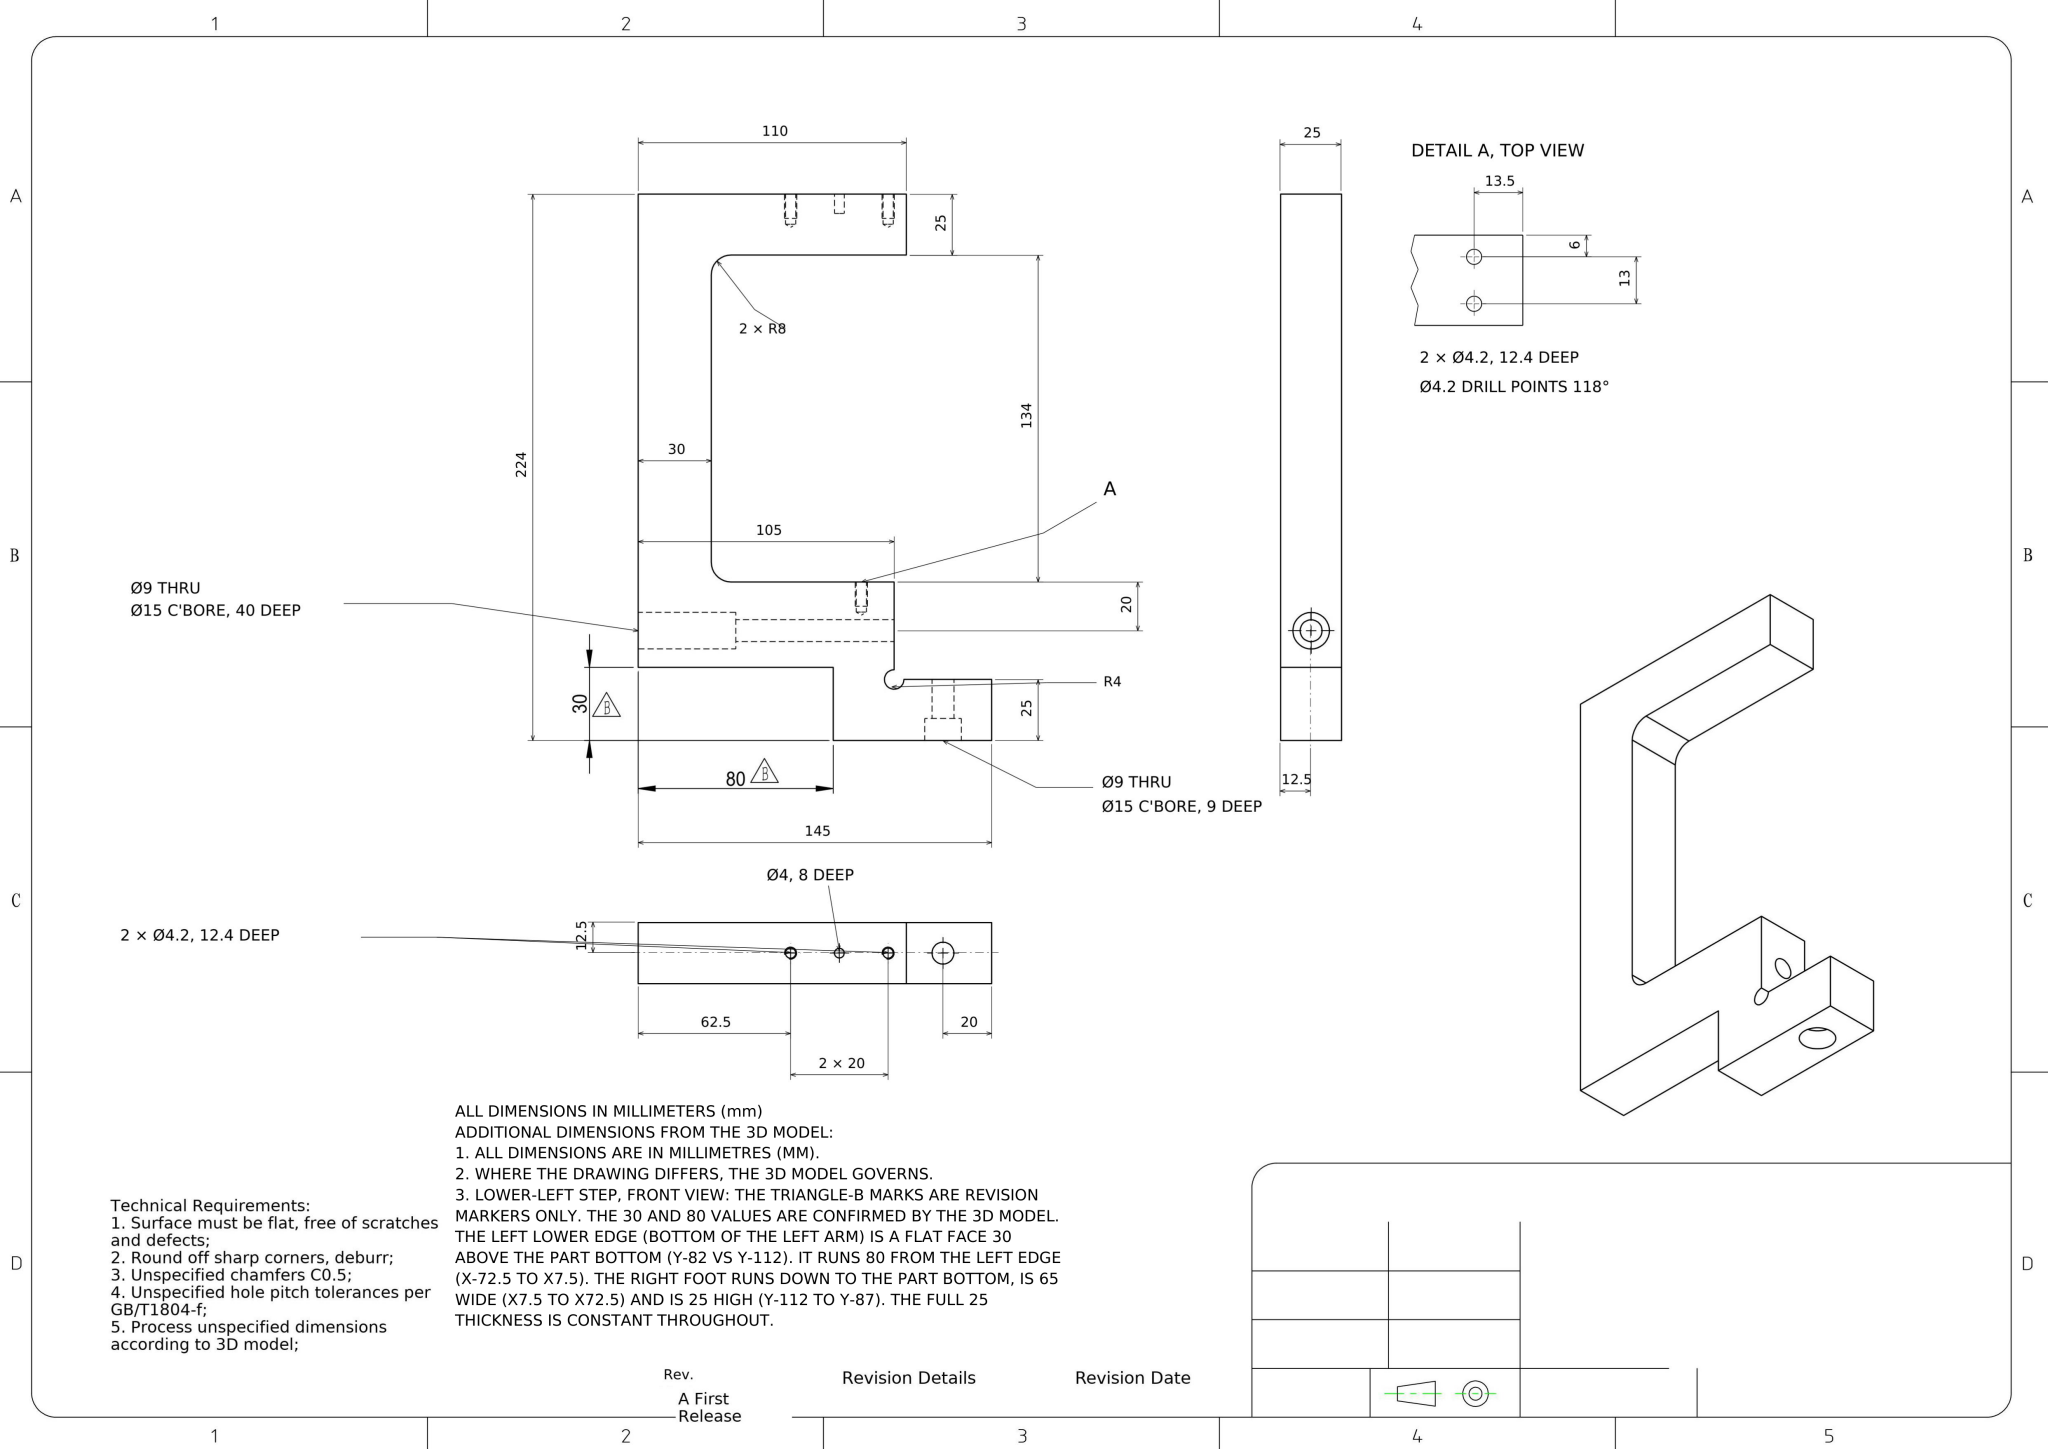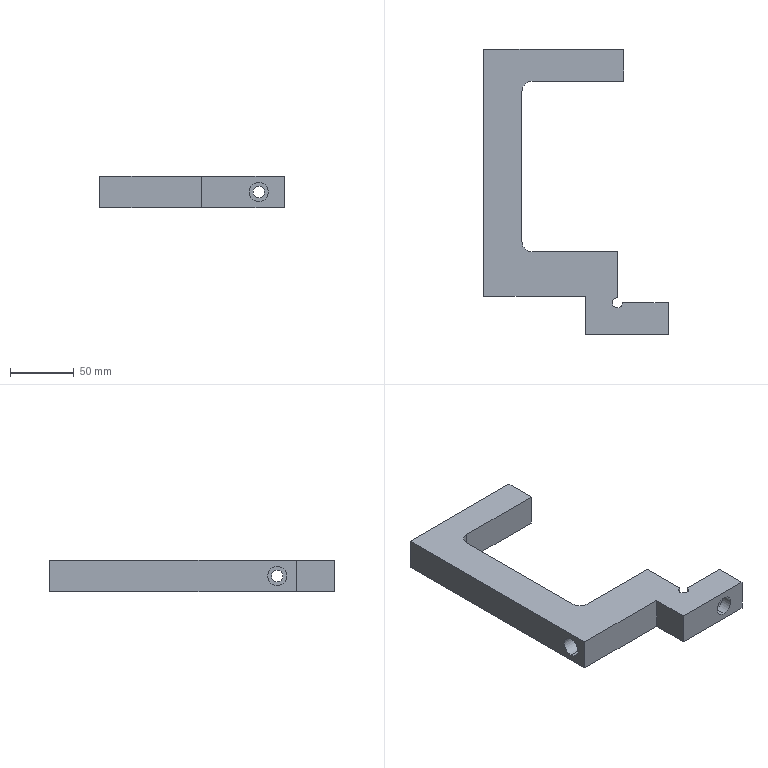Part | NX | mm | Dual-Leg Rectangular Frame Bracket | 1 solid | 47 faces | box 145 x 224 x 25 mm | volume 289996 mm3 | cylinder 22 | plane 17 | cone 8 | commonest cylinder face diameters 4.2 x8 15 x4 9 x4 8 x2 4 x2 16 x2